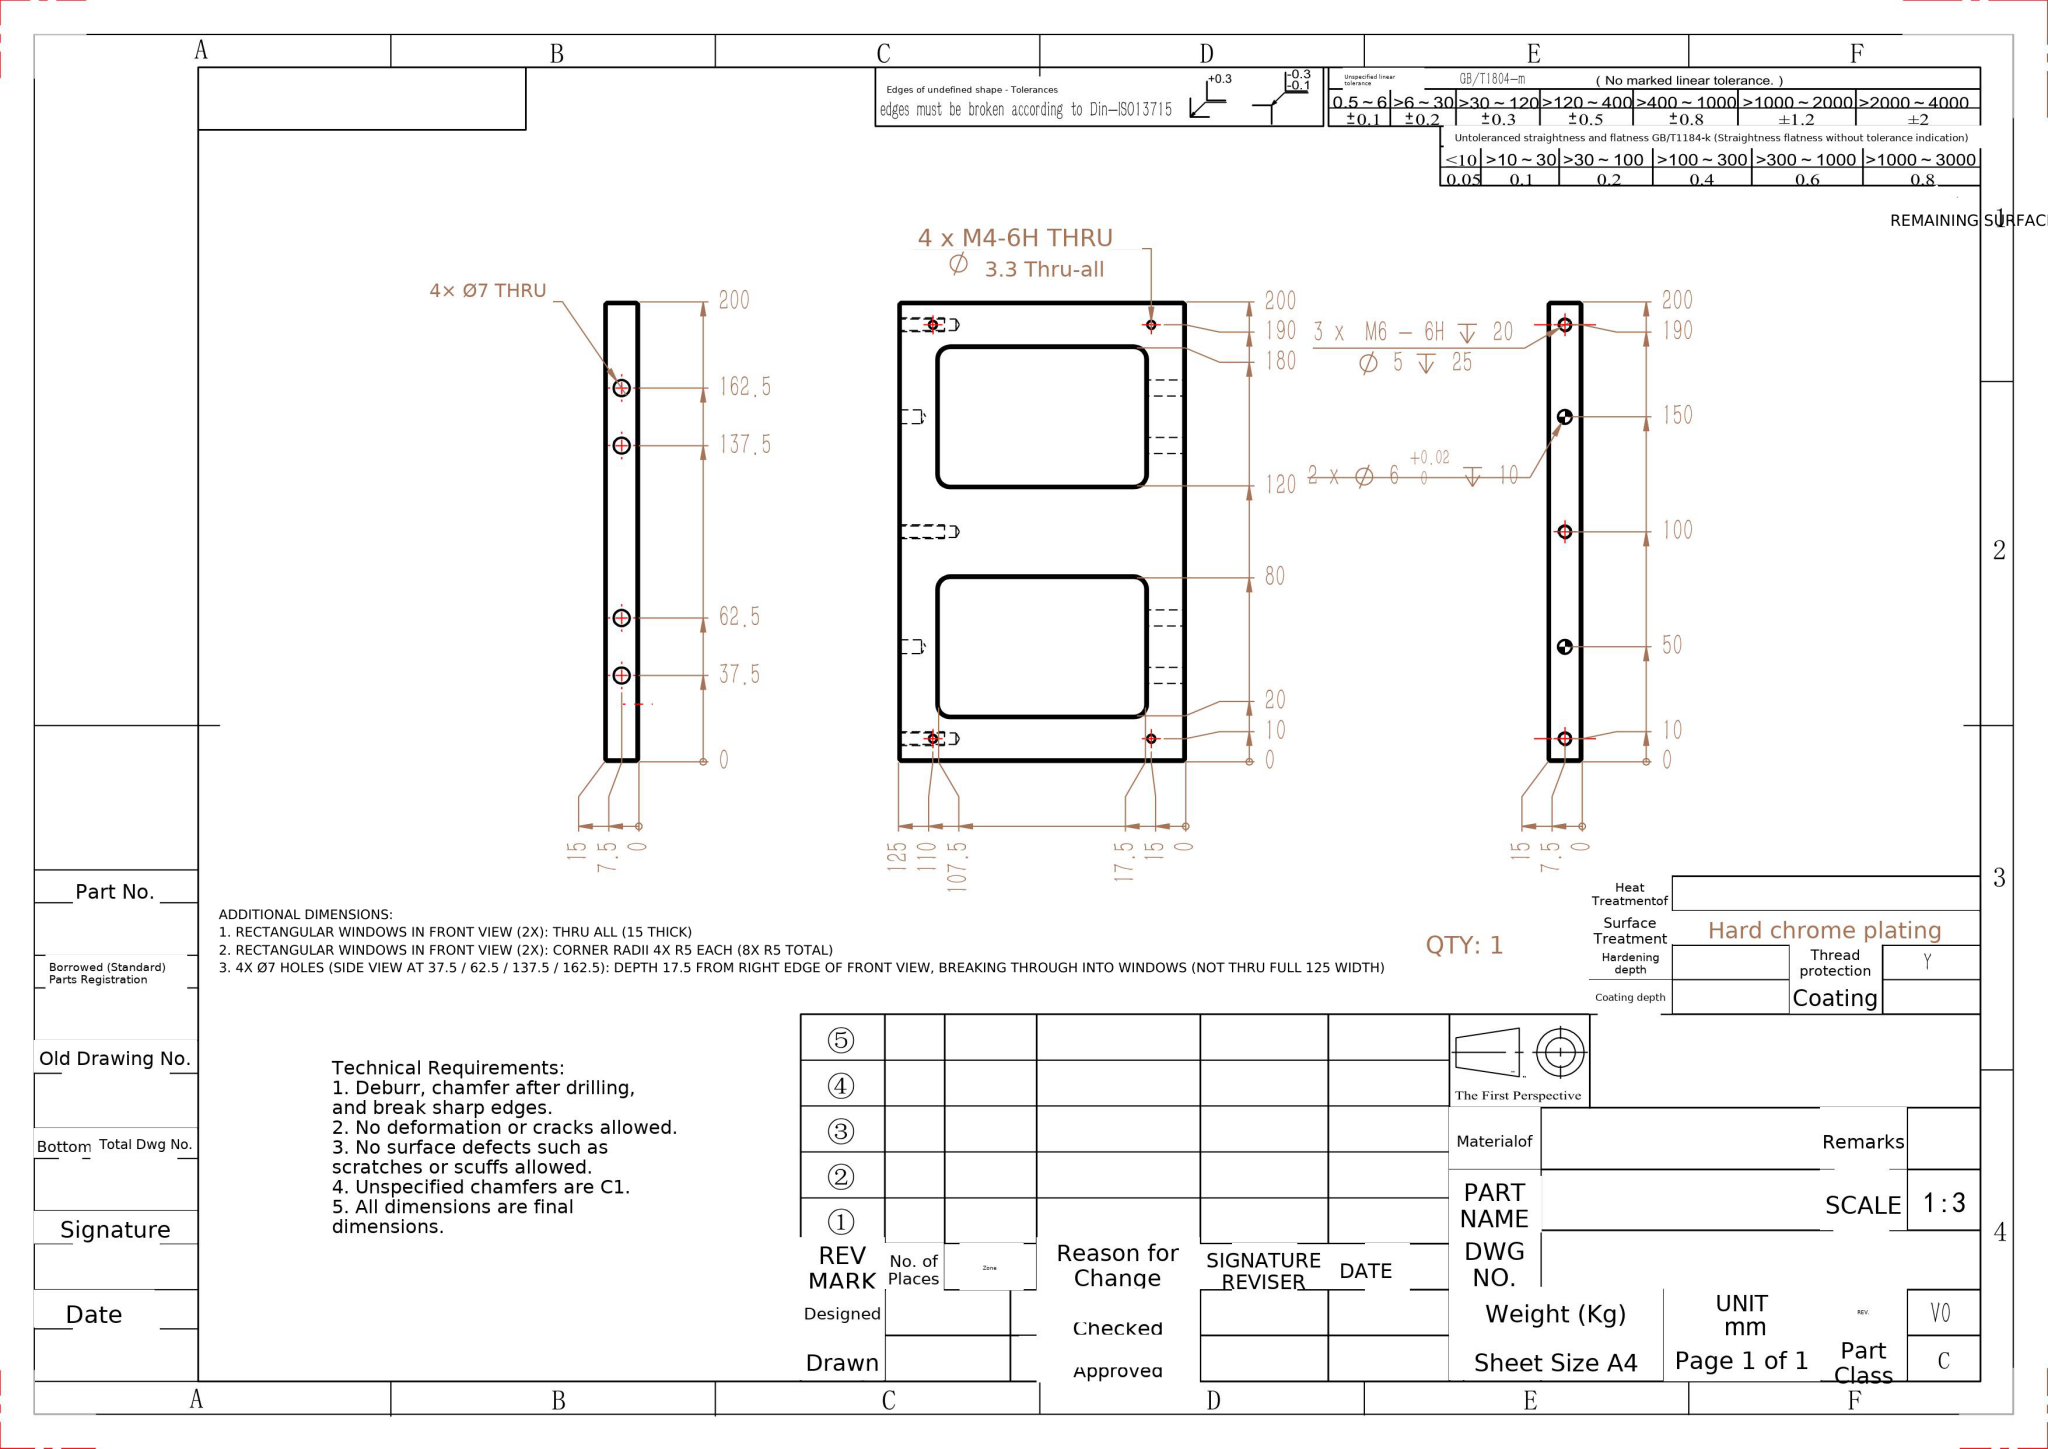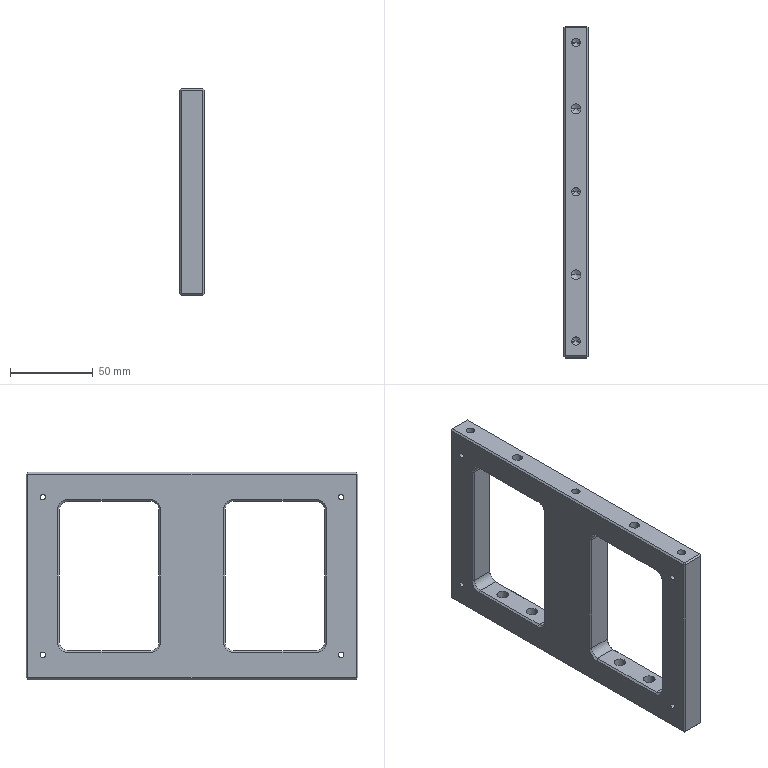Part | NX | mm | 1 solid | 114 faces | box 15 x 200 x 125 mm | volume 207154 mm3 | plane 50 | cylinder 38 | cone 26 | commonest cylinder face diameters 3.3 x12 7 x8 10 x8 5 x6 6 x4